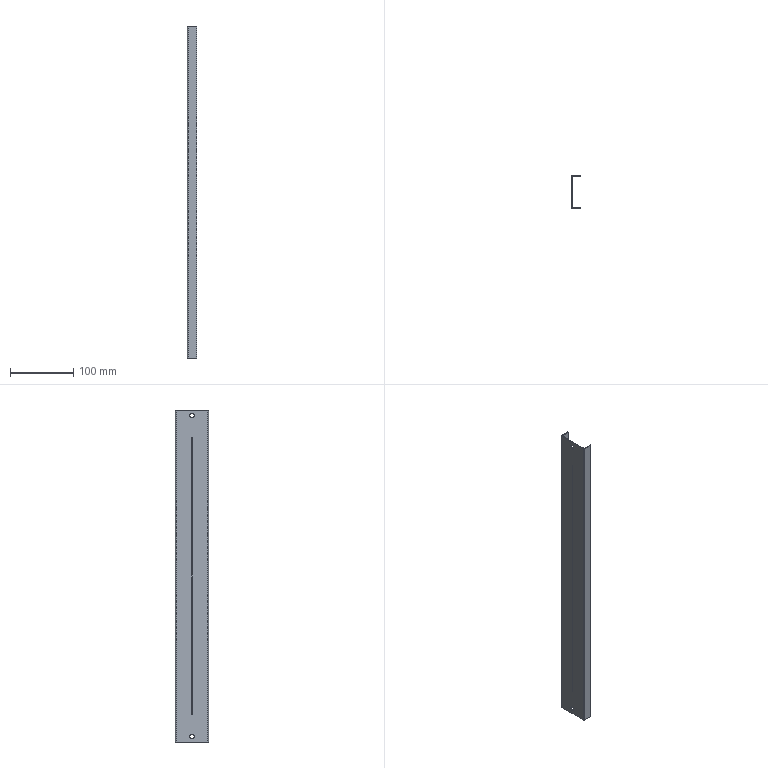Component | SolidWorks | FilmConnectionPlate-1 | 1 solid | 20 faces | box 15 x 52 x 523 mm | volume 60701 mm3 | plane 12 | cylinder 8 | commonest cylinder face diameters 7 x4 3 x2 1 x2
build123d program:
from build123d import *

# Parameters (mm, degrees)
BOSS_EXTRUDE1_DEPTH      = 523
SKETCH2_W                = 13.5
SKETCH2_H                = 49
CUT_EXTRUDE1_DEPTH       = 524.861
CUT_EXTRUDE2_DEPTH       = 264.136
F_7_0_7_DIAMETER_HOLE1_D = 7


with BuildPart() as part:
    # Sketch1 → Boss-Extrude1 (new body)
    with BuildSketch(Plane(origin=(0, 0, -261.5), x_dir=(-1, 0, 0), z_dir=(0, 0, -1))):
        with BuildLine():
            Line((1.5, -26), (15, -26))
            Line((15, -26), (15, 26))
            Line((15, 26), (1.5, 26))
            ThreePointArc((1.5, 26), (0.4393, 25.561), (0, 24.5))
            Line((0, 24.5), (0, -24.5))
            ThreePointArc((0, -24.5), (0.4393, -25.561), (1.5, -26))
        make_face()
    extrude(amount=-BOSS_EXTRUDE1_DEPTH)

    # Sketch2 → Cut-Extrude1 (cut, through all)
    with BuildSketch(Plane.XY.offset(261.5)):
        with Locations((-8.25, 0)):
            Rectangle(SKETCH2_W, SKETCH2_H)
    extrude(amount=-CUT_EXTRUDE1_DEPTH, mode=Mode.SUBTRACT)

    # Sketch3 → Cut-Extrude2 (cut, through all)
    with BuildSketch(Plane.ZY.offset(1.5)):
        with BuildLine():
            Line((217.5, 0.5), (-217.5, 0.5))
            ThreePointArc((-217.5, 0.5), (-218, 0), (-217.5, -0.5))
            Line((-217.5, -0.5), (217.5, -0.5))
            ThreePointArc((217.5, -0.5), (218, 0), (217.5, 0.5))
        make_face()
    extrude(amount=-CUT_EXTRUDE2_DEPTH, mode=Mode.SUBTRACT)

    # 7.0 _7_ Diameter Hole1 (through all)
    with Locations(Plane.ZY.offset(1.5)):
        with Locations((-252.5, 0), (252.5, 0)):
            Hole(F_7_0_7_DIAMETER_HOLE1_D / 2)


solid = part.part

# Placed as in the assembly
solid = solid.moved(Location((-376.5, 336, 0), (-180, 0, 180)))
STEP:
#1=CARTESIAN_POINT('',(-14.823,13.228,-10.079));
#2=VERTEX_POINT('',#1);
#3=CARTESIAN_POINT('',(-14.823,13.228,-9.803));
#4=VERTEX_POINT('',#3);
#5=CARTESIAN_POINT('',(-14.823,13.228,-9.941));
#6=DIRECTION('',(1.,0.,-0.));
#7=DIRECTION('',(0.,0.,1.));
#8=AXIS2_PLACEMENT_3D('',#5,#6,#7);
#9=CIRCLE('',#8,0.1378);
#10=EDGE_CURVE('',#2,#4,#9,.T.);
#11=ORIENTED_EDGE('',*,*,#10,.F.);
#12=CARTESIAN_POINT('',(-14.764,13.228,-10.079));
#13=VERTEX_POINT('',#12);
#14=CARTESIAN_POINT('',(-14.764,13.228,-10.079));
#15=DIRECTION('',(1.,0.,-0.));
#16=VECTOR('',#15,39.37);
#17=LINE('',#14,#16);
#18=EDGE_CURVE('',#2,#13,#17,.T.);
#19=ORIENTED_EDGE('',*,*,#18,.T.);
#20=CARTESIAN_POINT('',(-14.764,13.228,-9.803));
#21=VERTEX_POINT('',#20);
#22=CARTESIAN_POINT('',(-14.764,13.228,-9.941));
#23=DIRECTION('',(1.,0.,-0.));
#24=DIRECTION('',(0.,0.,1.));
#25=AXIS2_PLACEMENT_3D('',#22,#23,#24);
#26=CIRCLE('',#25,0.1378);
#27=EDGE_CURVE('',#13,#21,#26,.T.);
#28=ORIENTED_EDGE('',*,*,#27,.T.);
#29=CARTESIAN_POINT('',(-14.764,13.228,-9.803));
#30=DIRECTION('',(1.,0.,-0.));
#31=VECTOR('',#30,39.37);
#32=LINE('',#29,#31);
#33=EDGE_CURVE('',#4,#21,#32,.T.);
#34=ORIENTED_EDGE('',*,*,#33,.F.);
#35=EDGE_LOOP('',(#11,#19,#28,#34));
#36=FACE_OUTER_BOUND('',#35,.T.);
#37=CARTESIAN_POINT('',(-14.764,13.228,-9.941));
#38=DIRECTION('',(1.,0.,-0.));
#39=DIRECTION('',(0.,0.,1.));
#40=AXIS2_PLACEMENT_3D('',#37,#38,#39);
#41=CYLINDRICAL_SURFACE('',#40,0.1378);
#42=ADVANCED_FACE('',(#36),#41,.F.);
#43=CARTESIAN_POINT('',(-14.823,13.228,9.803));
#44=VERTEX_POINT('',#43);
#45=CARTESIAN_POINT('',(-14.823,13.228,10.079));
#46=VERTEX_POINT('',#45);
#47=CARTESIAN_POINT('',(-14.823,13.228,9.941));
#48=DIRECTION('',(1.,0.,-0.));
#49=DIRECTION('',(0.,0.,1.));
#50=AXIS2_PLACEMENT_3D('',#47,#48,#49);
#51=CIRCLE('',#50,0.1378);
#52=EDGE_CURVE('',#44,#46,#51,.T.);
#53=ORIENTED_EDGE('',*,*,#52,.F.);
#54=CARTESIAN_POINT('',(-14.764,13.228,9.803));
#55=VERTEX_POINT('',#54);
#56=CARTESIAN_POINT('',(-14.764,13.228,9.803));
#57=DIRECTION('',(1.,0.,-0.));
#58=VECTOR('',#57,39.37);
#59=LINE('',#56,#58);
#60=EDGE_CURVE('',#44,#55,#59,.T.);
#61=ORIENTED_EDGE('',*,*,#60,.T.);
#62=CARTESIAN_POINT('',(-14.764,13.228,10.079));
#63=VERTEX_POINT('',#62);
#64=CARTESIAN_POINT('',(-14.764,13.228,9.941));
#65=DIRECTION('',(1.,0.,-0.));
#66=DIRECTION('',(0.,0.,1.));
#67=AXIS2_PLACEMENT_3D('',#64,#65,#66);
#68=CIRCLE('',#67,0.1378);
#69=EDGE_CURVE('',#55,#63,#68,.T.);
#70=ORIENTED_EDGE('',*,*,#69,.T.);
#71=CARTESIAN_POINT('',(-14.764,13.228,10.079));
#72=DIRECTION('',(1.,0.,-0.));
#73=VECTOR('',#72,39.37);
#74=LINE('',#71,#73);
#75=EDGE_CURVE('',#46,#63,#74,.T.);
#76=ORIENTED_EDGE('',*,*,#75,.F.);
#77=EDGE_LOOP('',(#53,#61,#70,#76));
#78=FACE_OUTER_BOUND('',#77,.T.);
#79=CARTESIAN_POINT('',(-14.764,13.228,9.941));
#80=DIRECTION('',(1.,0.,-0.));
#81=DIRECTION('',(0.,0.,1.));
#82=AXIS2_PLACEMENT_3D('',#79,#80,#81);
#83=CYLINDRICAL_SURFACE('',#82,0.1378);
#84=ADVANCED_FACE('',(#78),#83,.F.);
#85=CARTESIAN_POINT('',(-14.232,12.264,-10.295));
#86=VERTEX_POINT('',#85);
#87=CARTESIAN_POINT('',(-14.232,12.264,10.295));
#88=VERTEX_POINT('',#87);
#89=CARTESIAN_POINT('',(-14.232,12.264,-10.295));
#90=DIRECTION('',(0.,0.,1.));
#91=VECTOR('',#90,39.37);
#92=LINE('',#89,#91);
#93=EDGE_CURVE('',#86,#88,#92,.T.);
#94=ORIENTED_EDGE('',*,*,#93,.T.);
#95=CARTESIAN_POINT('',(-14.232,12.205,10.295));
#96=VERTEX_POINT('',#95);
#97=CARTESIAN_POINT('',(-14.232,14.252,10.295));
#98=DIRECTION('',(0.,-1.,0.));
#99=VECTOR('',#98,39.37);
#100=LINE('',#97,#99);
#101=EDGE_CURVE('',#88,#96,#100,.T.);
#102=ORIENTED_EDGE('',*,*,#101,.T.);
#103=CARTESIAN_POINT('',(-14.232,12.205,-10.295));
#104=VERTEX_POINT('',#103);
#105=CARTESIAN_POINT('',(-14.232,12.205,10.295));
#106=DIRECTION('',(-0.,-0.,-1.));
#107=VECTOR('',#106,39.37);
#108=LINE('',#105,#107);
#109=EDGE_CURVE('',#96,#104,#108,.T.);
#110=ORIENTED_EDGE('',*,*,#109,.T.);
#111=CARTESIAN_POINT('',(-14.232,14.252,-10.295));
#112=DIRECTION('',(0.,-1.,0.));
#113=VECTOR('',#112,39.37);
#114=LINE('',#111,#113);
#115=EDGE_CURVE('',#86,#104,#114,.T.);
#116=ORIENTED_EDGE('',*,*,#115,.F.);
#117=EDGE_LOOP('',(#94,#102,#110,#116));
#118=FACE_OUTER_BOUND('',#117,.T.);
#119=CARTESIAN_POINT('',(-14.232,14.252,10.295));
#120=DIRECTION('',(1.,0.,-0.));
#121=DIRECTION('',(0.,0.,1.));
#122=AXIS2_PLACEMENT_3D('',#119,#120,#121);
#123=PLANE('',#122);
#124=ADVANCED_FACE('',(#118),#123,.T.);
#125=CARTESIAN_POINT('',(-14.823,14.193,-10.295));
#126=VERTEX_POINT('',#125);
#127=CARTESIAN_POINT('',(-14.764,14.252,-10.295));
#128=VERTEX_POINT('',#127);
#129=CARTESIAN_POINT('',(-14.764,14.193,-10.295));
#130=DIRECTION('',(-0.,-0.,-1.));
#131=DIRECTION('',(1.,0.,0.));
#132=AXIS2_PLACEMENT_3D('',#129,#130,#131);
#133=CIRCLE('',#132,0.05906);
#134=EDGE_CURVE('',#126,#128,#133,.T.);
#135=ORIENTED_EDGE('',*,*,#134,.F.);
#136=CARTESIAN_POINT('',(-14.823,14.193,10.295));
#137=VERTEX_POINT('',#136);
#138=CARTESIAN_POINT('',(-14.823,14.193,10.295));
#139=DIRECTION('',(-0.,-0.,-1.));
#140=VECTOR('',#139,39.37);
#141=LINE('',#138,#140);
#142=EDGE_CURVE('',#137,#126,#141,.T.);
#143=ORIENTED_EDGE('',*,*,#142,.F.);
#144=CARTESIAN_POINT('',(-14.764,14.252,10.295));
#145=VERTEX_POINT('',#144);
#146=CARTESIAN_POINT('',(-14.764,14.193,10.295));
#147=DIRECTION('',(-0.,-0.,-1.));
#148=DIRECTION('',(1.,0.,0.));
#149=AXIS2_PLACEMENT_3D('',#146,#147,#148);
#150=CIRCLE('',#149,0.05906);
#151=EDGE_CURVE('',#137,#145,#150,.T.);
#152=ORIENTED_EDGE('',*,*,#151,.T.);
#153=CARTESIAN_POINT('',(-14.764,14.252,10.295));
#154=DIRECTION('',(-0.,-0.,-1.));
#155=VECTOR('',#154,39.37);
#156=LINE('',#153,#155);
#157=EDGE_CURVE('',#145,#128,#156,.T.);
#158=ORIENTED_EDGE('',*,*,#157,.T.);
#159=EDGE_LOOP('',(#135,#143,#152,#158));
#160=FACE_OUTER_BOUND('',#159,.T.);
#161=CARTESIAN_POINT('',(-14.764,14.193,10.295));
#162=DIRECTION('',(-0.,-0.,-1.));
#163=DIRECTION('',(1.,0.,0.));
#164=AXIS2_PLACEMENT_3D('',#161,#162,#163);
#165=CYLINDRICAL_SURFACE('',#164,0.05906);
#166=ADVANCED_FACE('',(#160),#165,.T.);
#167=CARTESIAN_POINT('',(-14.823,13.228,-9.941));
#168=DIRECTION('',(1.,0.,-0.));
#169=DIRECTION('',(0.,0.,1.));
#170=AXIS2_PLACEMENT_3D('',#167,#168,#169);
#171=CIRCLE('',#170,0.1378);
#172=EDGE_CURVE('',#4,#2,#171,.T.);
#173=ORIENTED_EDGE('',*,*,#172,.T.);
#174=ORIENTED_EDGE('',*,*,#10,.T.);
#175=EDGE_LOOP('',(#173,#174));
#176=FACE_BOUND('',#175,.T.);
#177=CARTESIAN_POINT('',(-14.823,13.228,9.941));
#178=DIRECTION('',(1.,0.,-0.));
#179=DIRECTION('',(0.,0.,1.));
#180=AXIS2_PLACEMENT_3D('',#177,#178,#179);
#181=CIRCLE('',#180,0.1378);
#182=EDGE_CURVE('',#46,#44,#181,.T.);
#183=ORIENTED_EDGE('',*,*,#182,.T.);
#184=ORIENTED_EDGE('',*,*,#52,.T.);
#185=EDGE_LOOP('',(#183,#184));
#186=FACE_BOUND('',#185,.T.);
#187=CARTESIAN_POINT('',(-14.823,13.248,8.563));
#188=VERTEX_POINT('',#187);
#189=CARTESIAN_POINT('',(-14.823,13.209,8.563));
#190=VERTEX_POINT('',#189);
#191=CARTESIAN_POINT('',(-14.823,13.228,8.563));
#192=DIRECTION('',(1.,0.,-0.));
#193=DIRECTION('',(0.,1.,0.));
#194=AXIS2_PLACEMENT_3D('',#191,#192,#193);
#195=CIRCLE('',#194,0.01969);
#196=EDGE_CURVE('',#188,#190,#195,.T.);
#197=ORIENTED_EDGE('',*,*,#196,.T.);
#198=CARTESIAN_POINT('',(-14.823,13.209,-8.563));
#199=VERTEX_POINT('',#198);
#200=CARTESIAN_POINT('',(-14.823,13.209,8.563));
#201=DIRECTION('',(-0.,-0.,-1.));
#202=VECTOR('',#201,39.37);
#203=LINE('',#200,#202);
#204=EDGE_CURVE('',#190,#199,#203,.T.);
#205=ORIENTED_EDGE('',*,*,#204,.T.);
#206=CARTESIAN_POINT('',(-14.823,13.248,-8.563));
#207=VERTEX_POINT('',#206);
#208=CARTESIAN_POINT('',(-14.823,13.228,-8.563));
#209=DIRECTION('',(1.,0.,-0.));
#210=DIRECTION('',(0.,1.,0.));
#211=AXIS2_PLACEMENT_3D('',#208,#209,#210);
#212=CIRCLE('',#211,0.01969);
#213=EDGE_CURVE('',#199,#207,#212,.T.);
#214=ORIENTED_EDGE('',*,*,#213,.T.);
#215=CARTESIAN_POINT('',(-14.823,13.248,-8.563));
#216=DIRECTION('',(0.,0.,1.));
#217=VECTOR('',#216,39.37);
#218=LINE('',#215,#217);
#219=EDGE_CURVE('',#207,#188,#218,.T.);
#220=ORIENTED_EDGE('',*,*,#219,.T.);
#221=EDGE_LOOP('',(#197,#205,#214,#220));
#222=FACE_BOUND('',#221,.T.);
#223=CARTESIAN_POINT('',(-14.823,12.264,-10.295));
#224=VERTEX_POINT('',#223);
#225=CARTESIAN_POINT('',(-14.823,12.264,-10.295));
#226=DIRECTION('',(-0.,1.,-0.));
#227=VECTOR('',#226,39.37);
#228=LINE('',#225,#227);
#229=EDGE_CURVE('',#224,#126,#228,.T.);
#230=ORIENTED_EDGE('',*,*,#229,.F.);
#231=CARTESIAN_POINT('',(-14.823,12.264,10.295));
#232=VERTEX_POINT('',#231);
#233=CARTESIAN_POINT('',(-14.823,12.264,10.295));
#234=DIRECTION('',(-0.,-0.,-1.));
#235=VECTOR('',#234,39.37);
#236=LINE('',#233,#235);
#237=EDGE_CURVE('',#232,#224,#236,.T.);
#238=ORIENTED_EDGE('',*,*,#237,.F.);
#239=CARTESIAN_POINT('',(-14.823,12.264,10.295));
#240=DIRECTION('',(-0.,1.,-0.));
#241=VECTOR('',#240,39.37);
#242=LINE('',#239,#241);
#243=EDGE_CURVE('',#232,#137,#242,.T.);
#244=ORIENTED_EDGE('',*,*,#243,.T.);
#245=ORIENTED_EDGE('',*,*,#142,.T.);
#246=EDGE_LOOP('',(#230,#238,#244,#245));
#247=FACE_OUTER_BOUND('',#246,.T.);
#248=CARTESIAN_POINT('',(-14.823,12.264,10.295));
#249=DIRECTION('',(-1.,-0.,0.));
#250=DIRECTION('',(-0.,-0.,-1.));
#251=AXIS2_PLACEMENT_3D('',#248,#249,#250);
#252=PLANE('',#251);
#253=ADVANCED_FACE('',(#176,#186,#222,#247),#252,.T.);
#254=CARTESIAN_POINT('',(-14.764,12.205,-10.295));
#255=VERTEX_POINT('',#254);
#256=CARTESIAN_POINT('',(-14.764,12.264,-10.295));
#257=DIRECTION('',(-0.,-0.,-1.));
#258=DIRECTION('',(1.,0.,0.));
#259=AXIS2_PLACEMENT_3D('',#256,#257,#258);
#260=CIRCLE('',#259,0.05906);
#261=EDGE_CURVE('',#255,#224,#260,.T.);
#262=ORIENTED_EDGE('',*,*,#261,.F.);
#263=CARTESIAN_POINT('',(-14.764,12.205,10.295));
#264=VERTEX_POINT('',#263);
#265=CARTESIAN_POINT('',(-14.764,12.205,10.295));
#266=DIRECTION('',(-0.,-0.,-1.));
#267=VECTOR('',#266,39.37);
#268=LINE('',#265,#267);
#269=EDGE_CURVE('',#264,#255,#268,.T.);
#270=ORIENTED_EDGE('',*,*,#269,.F.);
#271=CARTESIAN_POINT('',(-14.764,12.264,10.295));
#272=DIRECTION('',(-0.,-0.,-1.));
#273=DIRECTION('',(1.,0.,0.));
#274=AXIS2_PLACEMENT_3D('',#271,#272,#273);
#275=CIRCLE('',#274,0.05906);
#276=EDGE_CURVE('',#264,#232,#275,.T.);
#277=ORIENTED_EDGE('',*,*,#276,.T.);
#278=ORIENTED_EDGE('',*,*,#237,.T.);
#279=EDGE_LOOP('',(#262,#270,#277,#278));
#280=FACE_OUTER_BOUND('',#279,.T.);
#281=CARTESIAN_POINT('',(-14.764,12.264,10.295));
#282=DIRECTION('',(-0.,-0.,-1.));
#283=DIRECTION('',(1.,0.,0.));
#284=AXIS2_PLACEMENT_3D('',#281,#282,#283);
#285=CYLINDRICAL_SURFACE('',#284,0.05906);
#286=ADVANCED_FACE('',(#280),#285,.T.);
#287=CARTESIAN_POINT('',(-14.232,12.205,-10.295));
#288=DIRECTION('',(-1.,-0.,0.));
#289=VECTOR('',#288,39.37);
#290=LINE('',#287,#289);
#291=EDGE_CURVE('',#104,#255,#290,.T.);
#292=ORIENTED_EDGE('',*,*,#291,.F.);
#293=ORIENTED_EDGE('',*,*,#109,.F.);
#294=CARTESIAN_POINT('',(-14.232,12.205,10.295));
#295=DIRECTION('',(-1.,-0.,0.));
#296=VECTOR('',#295,39.37);
#297=LINE('',#294,#296);
#298=EDGE_CURVE('',#96,#264,#297,.T.);
#299=ORIENTED_EDGE('',*,*,#298,.T.);
#300=ORIENTED_EDGE('',*,*,#269,.T.);
#301=EDGE_LOOP('',(#292,#293,#299,#300));
#302=FACE_OUTER_BOUND('',#301,.T.);
#303=CARTESIAN_POINT('',(-14.232,12.205,10.295));
#304=DIRECTION('',(0.,-1.,0.));
#305=DIRECTION('',(0.,0.,1.));
#306=AXIS2_PLACEMENT_3D('',#303,#304,#305);
#307=PLANE('',#306);
#308=ADVANCED_FACE('',(#302),#307,.T.);
#309=CARTESIAN_POINT('',(-14.232,14.193,-10.295));
#310=VERTEX_POINT('',#309);
#311=CARTESIAN_POINT('',(-14.232,14.193,10.295));
#312=VERTEX_POINT('',#311);
#313=CARTESIAN_POINT('',(-14.232,14.193,-10.295));
#314=DIRECTION('',(0.,0.,1.));
#315=VECTOR('',#314,39.37);
#316=LINE('',#313,#315);
#317=EDGE_CURVE('',#310,#312,#316,.T.);
#318=ORIENTED_EDGE('',*,*,#317,.F.);
#319=CARTESIAN_POINT('',(-14.232,14.252,-10.295));
#320=VERTEX_POINT('',#319);
#321=CARTESIAN_POINT('',(-14.232,14.252,-10.295));
#322=DIRECTION('',(0.,-1.,0.));
#323=VECTOR('',#322,39.37);
#324=LINE('',#321,#323);
#325=EDGE_CURVE('',#320,#310,#324,.T.);
#326=ORIENTED_EDGE('',*,*,#325,.F.);
#327=CARTESIAN_POINT('',(-14.232,14.252,10.295));
#328=VERTEX_POINT('',#327);
#329=CARTESIAN_POINT('',(-14.232,14.252,10.295));
#330=DIRECTION('',(-0.,-0.,-1.));
#331=VECTOR('',#330,39.37);
#332=LINE('',#329,#331);
#333=EDGE_CURVE('',#328,#320,#332,.T.);
#334=ORIENTED_EDGE('',*,*,#333,.F.);
#335=CARTESIAN_POINT('',(-14.232,14.252,10.295));
#336=DIRECTION('',(0.,-1.,0.));
#337=VECTOR('',#336,39.37);
#338=LINE('',#335,#337);
#339=EDGE_CURVE('',#328,#312,#338,.T.);
#340=ORIENTED_EDGE('',*,*,#339,.T.);
#341=EDGE_LOOP('',(#318,#326,#334,#340));
#342=FACE_OUTER_BOUND('',#341,.T.);
#343=CARTESIAN_POINT('',(-14.232,14.252,10.295));
#344=DIRECTION('',(1.,0.,-0.));
#345=DIRECTION('',(0.,0.,1.));
#346=AXIS2_PLACEMENT_3D('',#343,#344,#345);
#347=PLANE('',#346);
#348=ADVANCED_FACE('',(#342),#347,.T.);
#349=CARTESIAN_POINT('',(-14.764,14.252,-10.295));
#350=DIRECTION('',(1.,0.,-0.));
#351=VECTOR('',#350,39.37);
#352=LINE('',#349,#351);
#353=EDGE_CURVE('',#128,#320,#352,.T.);
#354=ORIENTED_EDGE('',*,*,#353,.F.);
#355=ORIENTED_EDGE('',*,*,#157,.F.);
#356=CARTESIAN_POINT('',(-14.764,14.252,10.295));
#357=DIRECTION('',(1.,0.,-0.));
#358=VECTOR('',#357,39.37);
#359=LINE('',#356,#358);
#360=EDGE_CURVE('',#145,#328,#359,.T.);
#361=ORIENTED_EDGE('',*,*,#360,.T.);
#362=ORIENTED_EDGE('',*,*,#333,.T.);
#363=EDGE_LOOP('',(#354,#355,#361,#362));
#364=FACE_OUTER_BOUND('',#363,.T.);
#365=CARTESIAN_POINT('',(-14.764,14.252,10.295));
#366=DIRECTION('',(-0.,1.,-0.));
#367=DIRECTION('',(-0.,-0.,-1.));
#368=AXIS2_PLACEMENT_3D('',#365,#366,#367);
#369=PLANE('',#368);
#370=ADVANCED_FACE('',(#364),#369,.T.);
#371=ORIENTED_EDGE('',*,*,#101,.F.);
#372=CARTESIAN_POINT('',(-14.764,12.264,10.295));
#373=VERTEX_POINT('',#372);
#374=CARTESIAN_POINT('',(-14.764,12.264,10.295));
#375=DIRECTION('',(1.,0.,-0.));
#376=VECTOR('',#375,39.37);
#377=LINE('',#374,#376);
#378=EDGE_CURVE('',#373,#88,#377,.T.);
#379=ORIENTED_EDGE('',*,*,#378,.F.);
#380=CARTESIAN_POINT('',(-14.764,14.193,10.295));
#381=VERTEX_POINT('',#380);
#382=CARTESIAN_POINT('',(-14.764,14.193,10.295));
#383=DIRECTION('',(0.,-1.,0.));
#384=VECTOR('',#383,39.37);
#385=LINE('',#382,#384);
#386=EDGE_CURVE('',#381,#373,#385,.T.);
#387=ORIENTED_EDGE('',*,*,#386,.F.);
#388=CARTESIAN_POINT('',(-14.232,14.193,10.295));
#389=DIRECTION('',(-1.,-0.,0.));
#390=VECTOR('',#389,39.37);
#391=LINE('',#388,#390);
#392=EDGE_CURVE('',#312,#381,#391,.T.);
#393=ORIENTED_EDGE('',*,*,#392,.F.);
#394=ORIENTED_EDGE('',*,*,#339,.F.);
#395=ORIENTED_EDGE('',*,*,#360,.F.);
#396=ORIENTED_EDGE('',*,*,#151,.F.);
#397=ORIENTED_EDGE('',*,*,#243,.F.);
#398=ORIENTED_EDGE('',*,*,#276,.F.);
#399=ORIENTED_EDGE('',*,*,#298,.F.);
#400=EDGE_LOOP('',(#371,#379,#387,#393,#394,#395,#396,#397,#398,#399));
#401=FACE_OUTER_BOUND('',#400,.T.);
#402=CARTESIAN_POINT('',(-14.764,14.193,10.295));
#403=DIRECTION('',(-0.,-0.,-1.));
#404=DIRECTION('',(1.,0.,-0.));
#405=AXIS2_PLACEMENT_3D('',#402,#403,#404);
#406=PLANE('',#405);
#407=ADVANCED_FACE('',(#401),#406,.F.);
#408=CARTESIAN_POINT('',(-14.764,12.264,-10.295));
#409=VERTEX_POINT('',#408);
#410=CARTESIAN_POINT('',(-14.764,12.264,-10.295));
#411=DIRECTION('',(1.,0.,-0.));
#412=VECTOR('',#411,39.37);
#413=LINE('',#410,#412);
#414=EDGE_CURVE('',#409,#86,#413,.T.);
#415=ORIENTED_EDGE('',*,*,#414,.T.);
#416=ORIENTED_EDGE('',*,*,#115,.T.);
#417=ORIENTED_EDGE('',*,*,#291,.T.);
#418=ORIENTED_EDGE('',*,*,#261,.T.);
#419=ORIENTED_EDGE('',*,*,#229,.T.);
#420=ORIENTED_EDGE('',*,*,#134,.T.);
#421=ORIENTED_EDGE('',*,*,#353,.T.);
#422=ORIENTED_EDGE('',*,*,#325,.T.);
#423=CARTESIAN_POINT('',(-14.764,14.193,-10.295));
#424=VERTEX_POINT('',#423);
#425=CARTESIAN_POINT('',(-14.232,14.193,-10.295));
#426=DIRECTION('',(-1.,-0.,0.));
#427=VECTOR('',#426,39.37);
#428=LINE('',#425,#427);
#429=EDGE_CURVE('',#310,#424,#428,.T.);
#430=ORIENTED_EDGE('',*,*,#429,.T.);
#431=CARTESIAN_POINT('',(-14.764,14.193,-10.295));
#432=DIRECTION('',(0.,-1.,0.));
#433=VECTOR('',#432,39.37);
#434=LINE('',#431,#433);
#435=EDGE_CURVE('',#424,#409,#434,.T.);
#436=ORIENTED_EDGE('',*,*,#435,.T.);
#437=EDGE_LOOP('',(#415,#416,#417,#418,#419,#420,#421,#422,#430,#436));
#438=FACE_OUTER_BOUND('',#437,.T.);
#439=CARTESIAN_POINT('',(-14.764,14.193,-10.295));
#440=DIRECTION('',(-0.,-0.,-1.));
#441=DIRECTION('',(1.,0.,-0.));
#442=AXIS2_PLACEMENT_3D('',#439,#440,#441);
#443=PLANE('',#442);
#444=ADVANCED_FACE('',(#438),#443,.T.);
#445=ORIENTED_EDGE('',*,*,#378,.T.);
#446=ORIENTED_EDGE('',*,*,#93,.F.);
#447=ORIENTED_EDGE('',*,*,#414,.F.);
#448=CARTESIAN_POINT('',(-14.764,12.264,-10.295));
#449=DIRECTION('',(0.,0.,1.));
#450=VECTOR('',#449,39.37);
#451=LINE('',#448,#450);
#452=EDGE_CURVE('',#409,#373,#451,.T.);
#453=ORIENTED_EDGE('',*,*,#452,.T.);
#454=EDGE_LOOP('',(#445,#446,#447,#453));
#455=FACE_OUTER_BOUND('',#454,.T.);
#456=CARTESIAN_POINT('',(-14.764,12.264,-10.295));
#457=DIRECTION('',(0.,-1.,0.));
#458=DIRECTION('',(0.,0.,1.));
#459=AXIS2_PLACEMENT_3D('',#456,#457,#458);
#460=PLANE('',#459);
#461=ADVANCED_FACE('',(#455),#460,.F.);
#462=CARTESIAN_POINT('',(-14.764,13.228,-9.941));
#463=DIRECTION('',(1.,0.,-0.));
#464=DIRECTION('',(0.,0.,1.));
#465=AXIS2_PLACEMENT_3D('',#462,#463,#464);
#466=CIRCLE('',#465,0.1378);
#467=EDGE_CURVE('',#21,#13,#466,.T.);
#468=ORIENTED_EDGE('',*,*,#467,.F.);
#469=ORIENTED_EDGE('',*,*,#27,.F.);
#470=EDGE_LOOP('',(#468,#469));
#471=FACE_BOUND('',#470,.T.);
#472=CARTESIAN_POINT('',(-14.764,13.228,9.941));
#473=DIRECTION('',(1.,0.,-0.));
#474=DIRECTION('',(0.,0.,1.));
#475=AXIS2_PLACEMENT_3D('',#472,#473,#474);
#476=CIRCLE('',#475,0.1378);
#477=EDGE_CURVE('',#63,#55,#476,.T.);
#478=ORIENTED_EDGE('',*,*,#477,.F.);
#479=ORIENTED_EDGE('',*,*,#69,.F.);
#480=EDGE_LOOP('',(#478,#479));
#481=FACE_BOUND('',#480,.T.);
#482=CARTESIAN_POINT('',(-14.764,13.209,8.563));
#483=VERTEX_POINT('',#482);
#484=CARTESIAN_POINT('',(-14.764,13.209,-8.563));
#485=VERTEX_POINT('',#484);
#486=CARTESIAN_POINT('',(-14.764,13.209,8.563));
#487=DIRECTION('',(-0.,-0.,-1.));
#488=VECTOR('',#487,39.37);
#489=LINE('',#486,#488);
#490=EDGE_CURVE('',#483,#485,#489,.T.);
#491=ORIENTED_EDGE('',*,*,#490,.F.);
#492=CARTESIAN_POINT('',(-14.764,13.248,8.563));
#493=VERTEX_POINT('',#492);
#494=CARTESIAN_POINT('',(-14.764,13.228,8.563));
#495=DIRECTION('',(1.,0.,-0.));
#496=DIRECTION('',(0.,1.,0.));
#497=AXIS2_PLACEMENT_3D('',#494,#495,#496);
#498=CIRCLE('',#497,0.01969);
#499=EDGE_CURVE('',#493,#483,#498,.T.);
#500=ORIENTED_EDGE('',*,*,#499,.F.);
#501=CARTESIAN_POINT('',(-14.764,13.248,-8.563));
#502=VERTEX_POINT('',#501);
#503=CARTESIAN_POINT('',(-14.764,13.248,-8.563));
#504=DIRECTION('',(0.,0.,1.));
#505=VECTOR('',#504,39.37);
#506=LINE('',#503,#505);
#507=EDGE_CURVE('',#502,#493,#506,.T.);
#508=ORIENTED_EDGE('',*,*,#507,.F.);
#509=CARTESIAN_POINT('',(-14.764,13.228,-8.563));
#510=DIRECTION('',(1.,0.,-0.));
#511=DIRECTION('',(0.,1.,0.));
#512=AXIS2_PLACEMENT_3D('',#509,#510,#511);
#513=CIRCLE('',#512,0.01969);
#514=EDGE_CURVE('',#485,#502,#513,.T.);
#515=ORIENTED_EDGE('',*,*,#514,.F.);
#516=EDGE_LOOP('',(#491,#500,#508,#515));
#517=FACE_BOUND('',#516,.T.);
#518=ORIENTED_EDGE('',*,*,#386,.T.);
#519=ORIENTED_EDGE('',*,*,#452,.F.);
#520=ORIENTED_EDGE('',*,*,#435,.F.);
#521=CARTESIAN_POINT('',(-14.764,14.193,-10.295));
#522=DIRECTION('',(0.,0.,1.));
#523=VECTOR('',#522,39.37);
#524=LINE('',#521,#523);
#525=EDGE_CURVE('',#424,#381,#524,.T.);
#526=ORIENTED_EDGE('',*,*,#525,.T.);
#527=EDGE_LOOP('',(#518,#519,#520,#526));
#528=FACE_OUTER_BOUND('',#527,.T.);
#529=CARTESIAN_POINT('',(-14.764,14.193,-10.295));
#530=DIRECTION('',(-1.,-0.,0.));
#531=DIRECTION('',(0.,-1.,0.));
#532=AXIS2_PLACEMENT_3D('',#529,#530,#531);
#533=PLANE('',#532);
#534=ADVANCED_FACE('',(#471,#481,#517,#528),#533,.F.);
#535=ORIENTED_EDGE('',*,*,#392,.T.);
#536=ORIENTED_EDGE('',*,*,#525,.F.);
#537=ORIENTED_EDGE('',*,*,#429,.F.);
#538=ORIENTED_EDGE('',*,*,#317,.T.);
#539=EDGE_LOOP('',(#535,#536,#537,#538));
#540=FACE_OUTER_BOUND('',#539,.T.);
#541=CARTESIAN_POINT('',(-14.232,14.193,-10.295));
#542=DIRECTION('',(-0.,1.,-0.));
#543=DIRECTION('',(-0.,-0.,-1.));
#544=AXIS2_PLACEMENT_3D('',#541,#542,#543);
#545=PLANE('',#544);
#546=ADVANCED_FACE('',(#540),#545,.F.);
#547=ORIENTED_EDGE('',*,*,#499,.T.);
#548=CARTESIAN_POINT('',(-14.823,13.209,8.563));
#549=DIRECTION('',(1.,0.,-0.));
#550=VECTOR('',#549,39.37);
#551=LINE('',#548,#550);
#552=EDGE_CURVE('',#190,#483,#551,.T.);
#553=ORIENTED_EDGE('',*,*,#552,.F.);
#554=ORIENTED_EDGE('',*,*,#196,.F.);
#555=CARTESIAN_POINT('',(-14.823,13.248,8.563));
#556=DIRECTION('',(1.,0.,-0.));
#557=VECTOR('',#556,39.37);
#558=LINE('',#555,#557);
#559=EDGE_CURVE('',#188,#493,#558,.T.);
#560=ORIENTED_EDGE('',*,*,#559,.T.);
#561=EDGE_LOOP('',(#547,#553,#554,#560));
#562=FACE_OUTER_BOUND('',#561,.T.);
#563=CARTESIAN_POINT('',(-14.823,13.228,8.563));
#564=DIRECTION('',(1.,0.,-0.));
#565=DIRECTION('',(0.,1.,0.));
#566=AXIS2_PLACEMENT_3D('',#563,#564,#565);
#567=CYLINDRICAL_SURFACE('',#566,0.01969);
#568=ADVANCED_FACE('',(#562),#567,.F.);
#569=ORIENTED_EDGE('',*,*,#507,.T.);
#570=ORIENTED_EDGE('',*,*,#559,.F.);
#571=ORIENTED_EDGE('',*,*,#219,.F.);
#572=CARTESIAN_POINT('',(-14.823,13.248,-8.563));
#573=DIRECTION('',(1.,0.,-0.));
#574=VECTOR('',#573,39.37);
#575=LINE('',#572,#574);
#576=EDGE_CURVE('',#207,#502,#575,.T.);
#577=ORIENTED_EDGE('',*,*,#576,.T.);
#578=EDGE_LOOP('',(#569,#570,#571,#577));
#579=FACE_OUTER_BOUND('',#578,.T.);
#580=CARTESIAN_POINT('',(-14.823,13.248,-8.563));
#581=DIRECTION('',(-0.,1.,-0.));
#582=DIRECTION('',(-0.,-0.,-1.));
#583=AXIS2_PLACEMENT_3D('',#580,#581,#582);
#584=PLANE('',#583);
#585=ADVANCED_FACE('',(#579),#584,.F.);
#586=ORIENTED_EDGE('',*,*,#514,.T.);
#587=ORIENTED_EDGE('',*,*,#576,.F.);
#588=ORIENTED_EDGE('',*,*,#213,.F.);
#589=CARTESIAN_POINT('',(-14.823,13.209,-8.563));
#590=DIRECTION('',(1.,0.,-0.));
#591=VECTOR('',#590,39.37);
#592=LINE('',#589,#591);
#593=EDGE_CURVE('',#199,#485,#592,.T.);
#594=ORIENTED_EDGE('',*,*,#593,.T.);
#595=EDGE_LOOP('',(#586,#587,#588,#594));
#596=FACE_OUTER_BOUND('',#595,.T.);
#597=CARTESIAN_POINT('',(-14.823,13.228,-8.563));
#598=DIRECTION('',(1.,0.,-0.));
#599=DIRECTION('',(0.,1.,0.));
#600=AXIS2_PLACEMENT_3D('',#597,#598,#599);
#601=CYLINDRICAL_SURFACE('',#600,0.01969);
#602=ADVANCED_FACE('',(#596),#601,.F.);
#603=ORIENTED_EDGE('',*,*,#490,.T.);
#604=ORIENTED_EDGE('',*,*,#593,.F.);
#605=ORIENTED_EDGE('',*,*,#204,.F.);
#606=ORIENTED_EDGE('',*,*,#552,.T.);
#607=EDGE_LOOP('',(#603,#604,#605,#606));
#608=FACE_OUTER_BOUND('',#607,.T.);
#609=CARTESIAN_POINT('',(-14.823,13.209,8.563));
#610=DIRECTION('',(0.,-1.,0.));
#611=DIRECTION('',(0.,0.,1.));
#612=AXIS2_PLACEMENT_3D('',#609,#610,#611);
#613=PLANE('',#612);
#614=ADVANCED_FACE('',(#608),#613,.F.);
#615=ORIENTED_EDGE('',*,*,#60,.F.);
#616=ORIENTED_EDGE('',*,*,#182,.F.);
#617=ORIENTED_EDGE('',*,*,#75,.T.);
#618=ORIENTED_EDGE('',*,*,#477,.T.);
#619=EDGE_LOOP('',(#615,#616,#617,#618));
#620=FACE_OUTER_BOUND('',#619,.T.);
#621=CARTESIAN_POINT('',(-14.764,13.228,9.941));
#622=DIRECTION('',(1.,0.,-0.));
#623=DIRECTION('',(0.,0.,1.));
#624=AXIS2_PLACEMENT_3D('',#621,#622,#623);
#625=CYLINDRICAL_SURFACE('',#624,0.1378);
#626=ADVANCED_FACE('',(#620),#625,.F.);
#627=ORIENTED_EDGE('',*,*,#18,.F.);
#628=ORIENTED_EDGE('',*,*,#172,.F.);
#629=ORIENTED_EDGE('',*,*,#33,.T.);
#630=ORIENTED_EDGE('',*,*,#467,.T.);
#631=EDGE_LOOP('',(#627,#628,#629,#630));
#632=FACE_OUTER_BOUND('',#631,.T.);
#633=CARTESIAN_POINT('',(-14.764,13.228,-9.941));
#634=DIRECTION('',(1.,0.,-0.));
#635=DIRECTION('',(0.,0.,1.));
#636=AXIS2_PLACEMENT_3D('',#633,#634,#635);
#637=CYLINDRICAL_SURFACE('',#636,0.1378);
#638=ADVANCED_FACE('',(#632),#637,.F.);
#639=CLOSED_SHELL('',(#42,#84,#124,#166,#253,#286,#308,#348,#370,#407,#444,#461,#534,#546,#568,#585,#602,#614,#626,#638));
#640=MANIFOLD_SOLID_BREP('',#639);
#641=CARTESIAN_POINT('',(0.,0.,0.));
#642=DIRECTION('',(0.,0.,1.));
#643=DIRECTION('',(1.,0.,0.));
#644=AXIS2_PLACEMENT_3D('',#641,#642,#643);
#645=(LENGTH_UNIT()NAMED_UNIT(*)SI_UNIT($,.METRE.));
#646=LENGTH_MEASURE_WITH_UNIT(LENGTH_MEASURE(0.0254),#645);
#647=DIMENSIONAL_EXPONENTS(1.,0.,0.,0.,0.,0.,0.);
#648=(CONVERSION_BASED_UNIT('',#646)LENGTH_UNIT()NAMED_UNIT(#647));
#649=UNCERTAINTY_MEASURE_WITH_UNIT(LENGTH_MEASURE(0.00001),#648,'','');
#650=(NAMED_UNIT(*)PLANE_ANGLE_UNIT()SI_UNIT($,.RADIAN.));
#651=(NAMED_UNIT(*)SI_UNIT($,.STERADIAN.)SOLID_ANGLE_UNIT());
#652=(GEOMETRIC_REPRESENTATION_CONTEXT(3)GLOBAL_UNCERTAINTY_ASSIGNED_CONTEXT((#649))GLOBAL_UNIT_ASSIGNED_CONTEXT((#648,#650,#651))REPRESENTATION_CONTEXT('',''));
#653=ADVANCED_BREP_SHAPE_REPRESENTATION('',(#640,#644),#652);
#654=COLOUR_RGB('',0.7922,0.8196,0.9333);
#655=FILL_AREA_STYLE_COLOUR('',#654);
#656=FILL_AREA_STYLE('',(#655));
#657=SURFACE_STYLE_FILL_AREA(#656);
#658=SURFACE_SIDE_STYLE('',(#657));
#659=SURFACE_STYLE_USAGE(.BOTH.,#658);
#660=PRESENTATION_STYLE_ASSIGNMENT((#659));
#661=STYLED_ITEM('',(#660),#640);
#662=(LENGTH_UNIT()NAMED_UNIT(*)SI_UNIT($,.METRE.));
#663=LENGTH_MEASURE_WITH_UNIT(LENGTH_MEASURE(0.0254),#662);
#664=DIMENSIONAL_EXPONENTS(1.,0.,0.,0.,0.,0.,0.);
#665=(CONVERSION_BASED_UNIT('',#663)LENGTH_UNIT()NAMED_UNIT(#664));
#666=UNCERTAINTY_MEASURE_WITH_UNIT(LENGTH_MEASURE(0.00001),#665,'','');
#667=(NAMED_UNIT(*)PLANE_ANGLE_UNIT()SI_UNIT($,.RADIAN.));
#668=(NAMED_UNIT(*)SI_UNIT($,.STERADIAN.)SOLID_ANGLE_UNIT());
#669=(GEOMETRIC_REPRESENTATION_CONTEXT(3)GLOBAL_UNCERTAINTY_ASSIGNED_CONTEXT((#666))GLOBAL_UNIT_ASSIGNED_CONTEXT((#665,#667,#668))REPRESENTATION_CONTEXT('',''));
#670=MECHANICAL_DESIGN_GEOMETRIC_PRESENTATION_REPRESENTATION('',(#661),#669);
#671=PRESENTATION_LAYER_ASSIGNMENT('','',(#661));